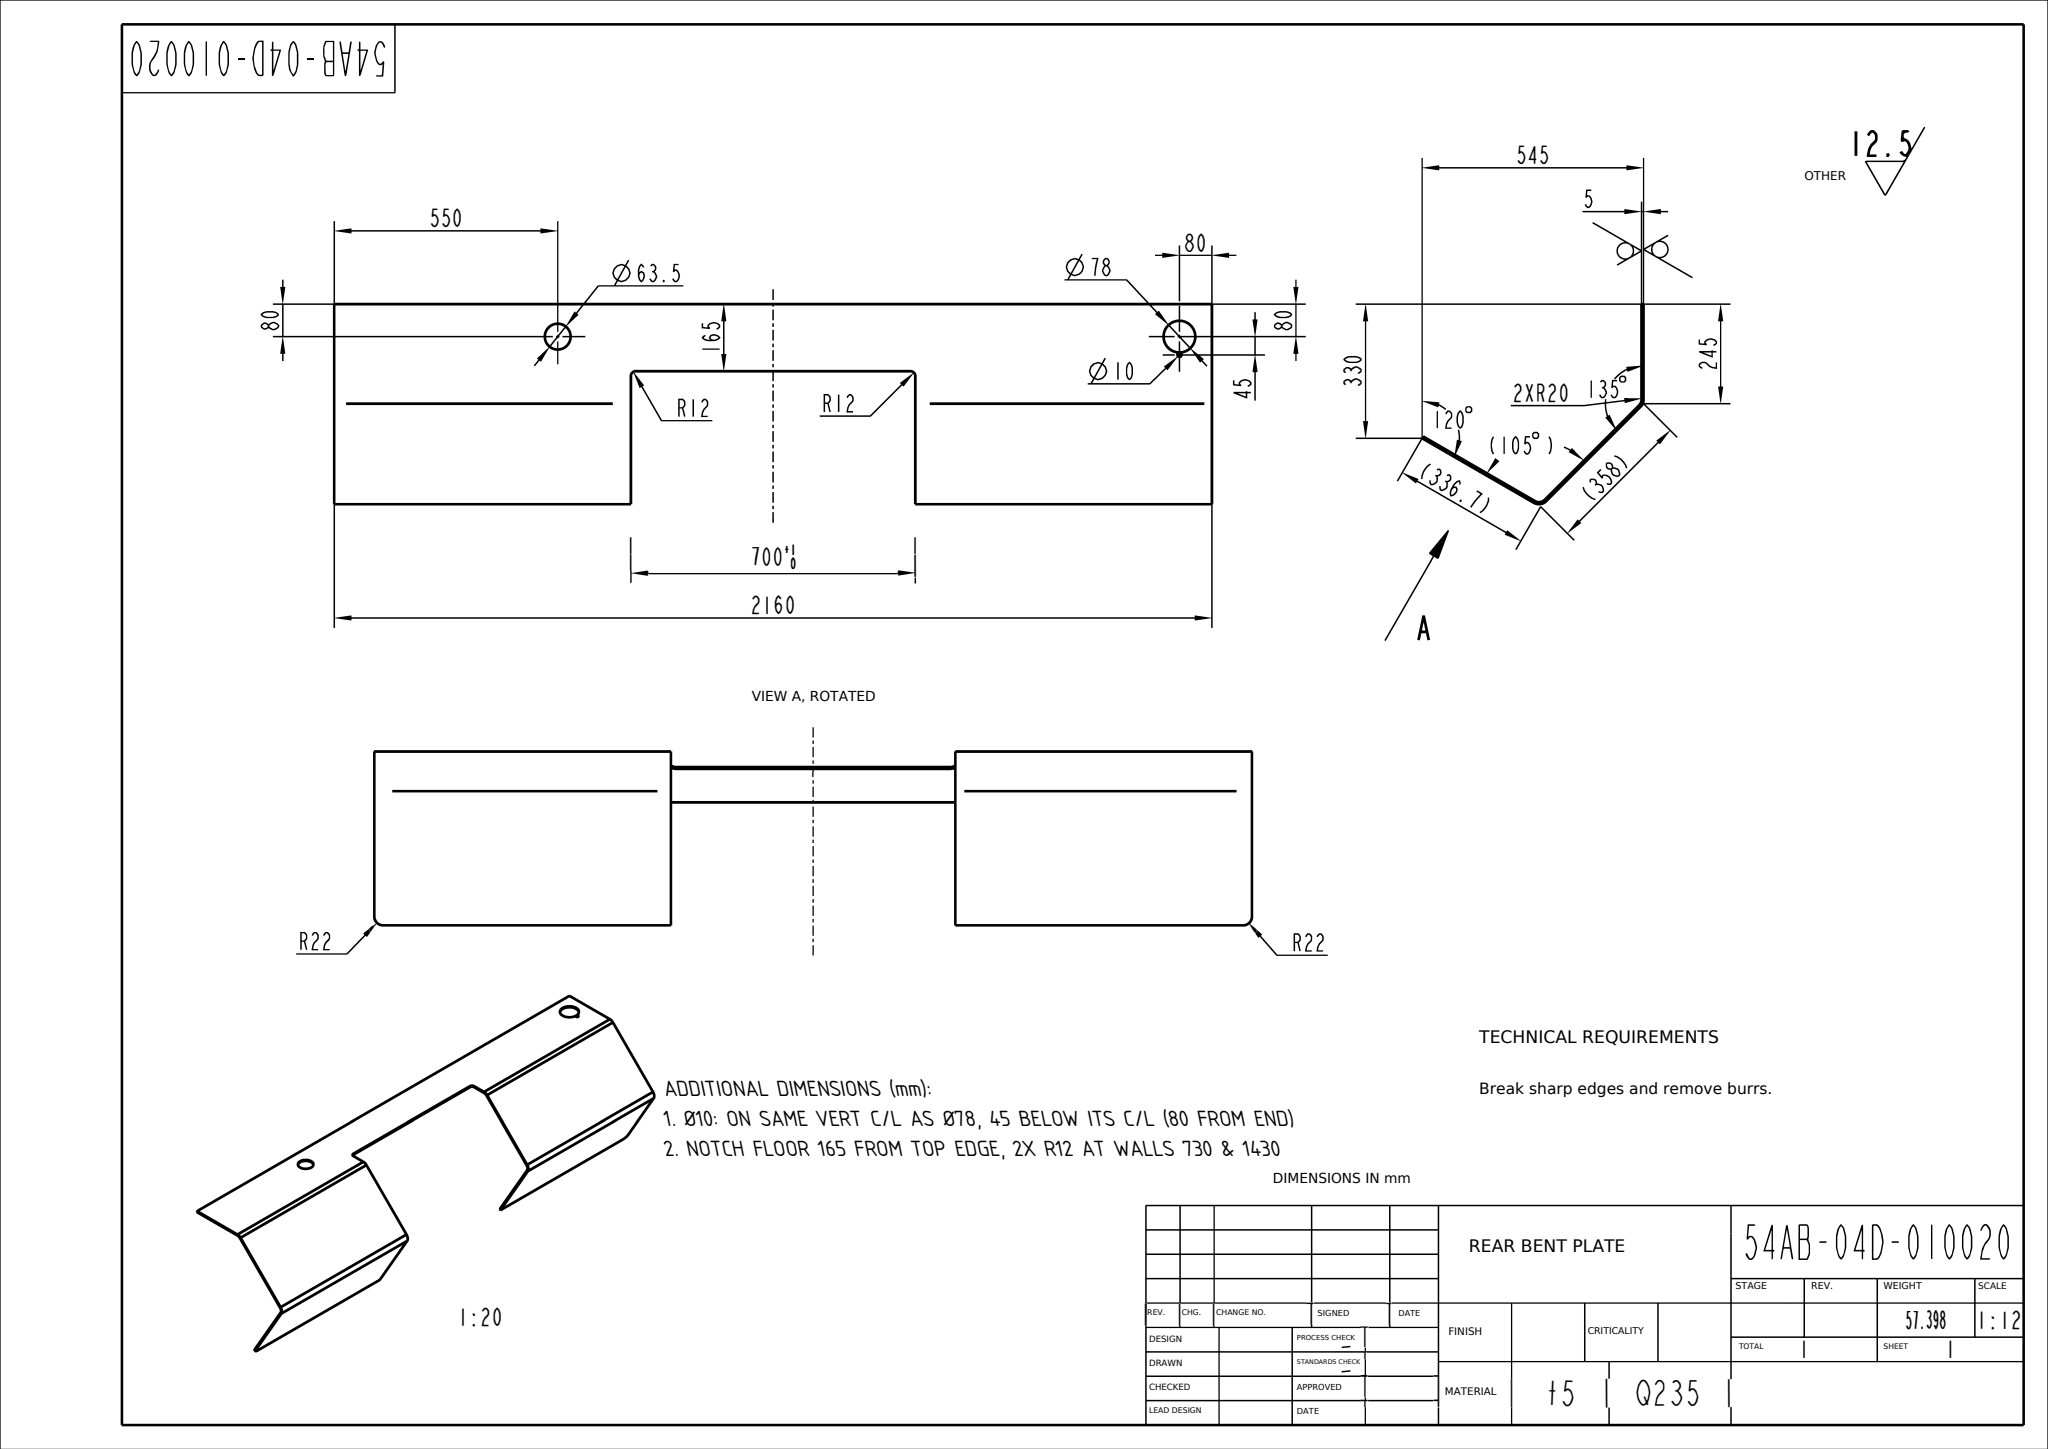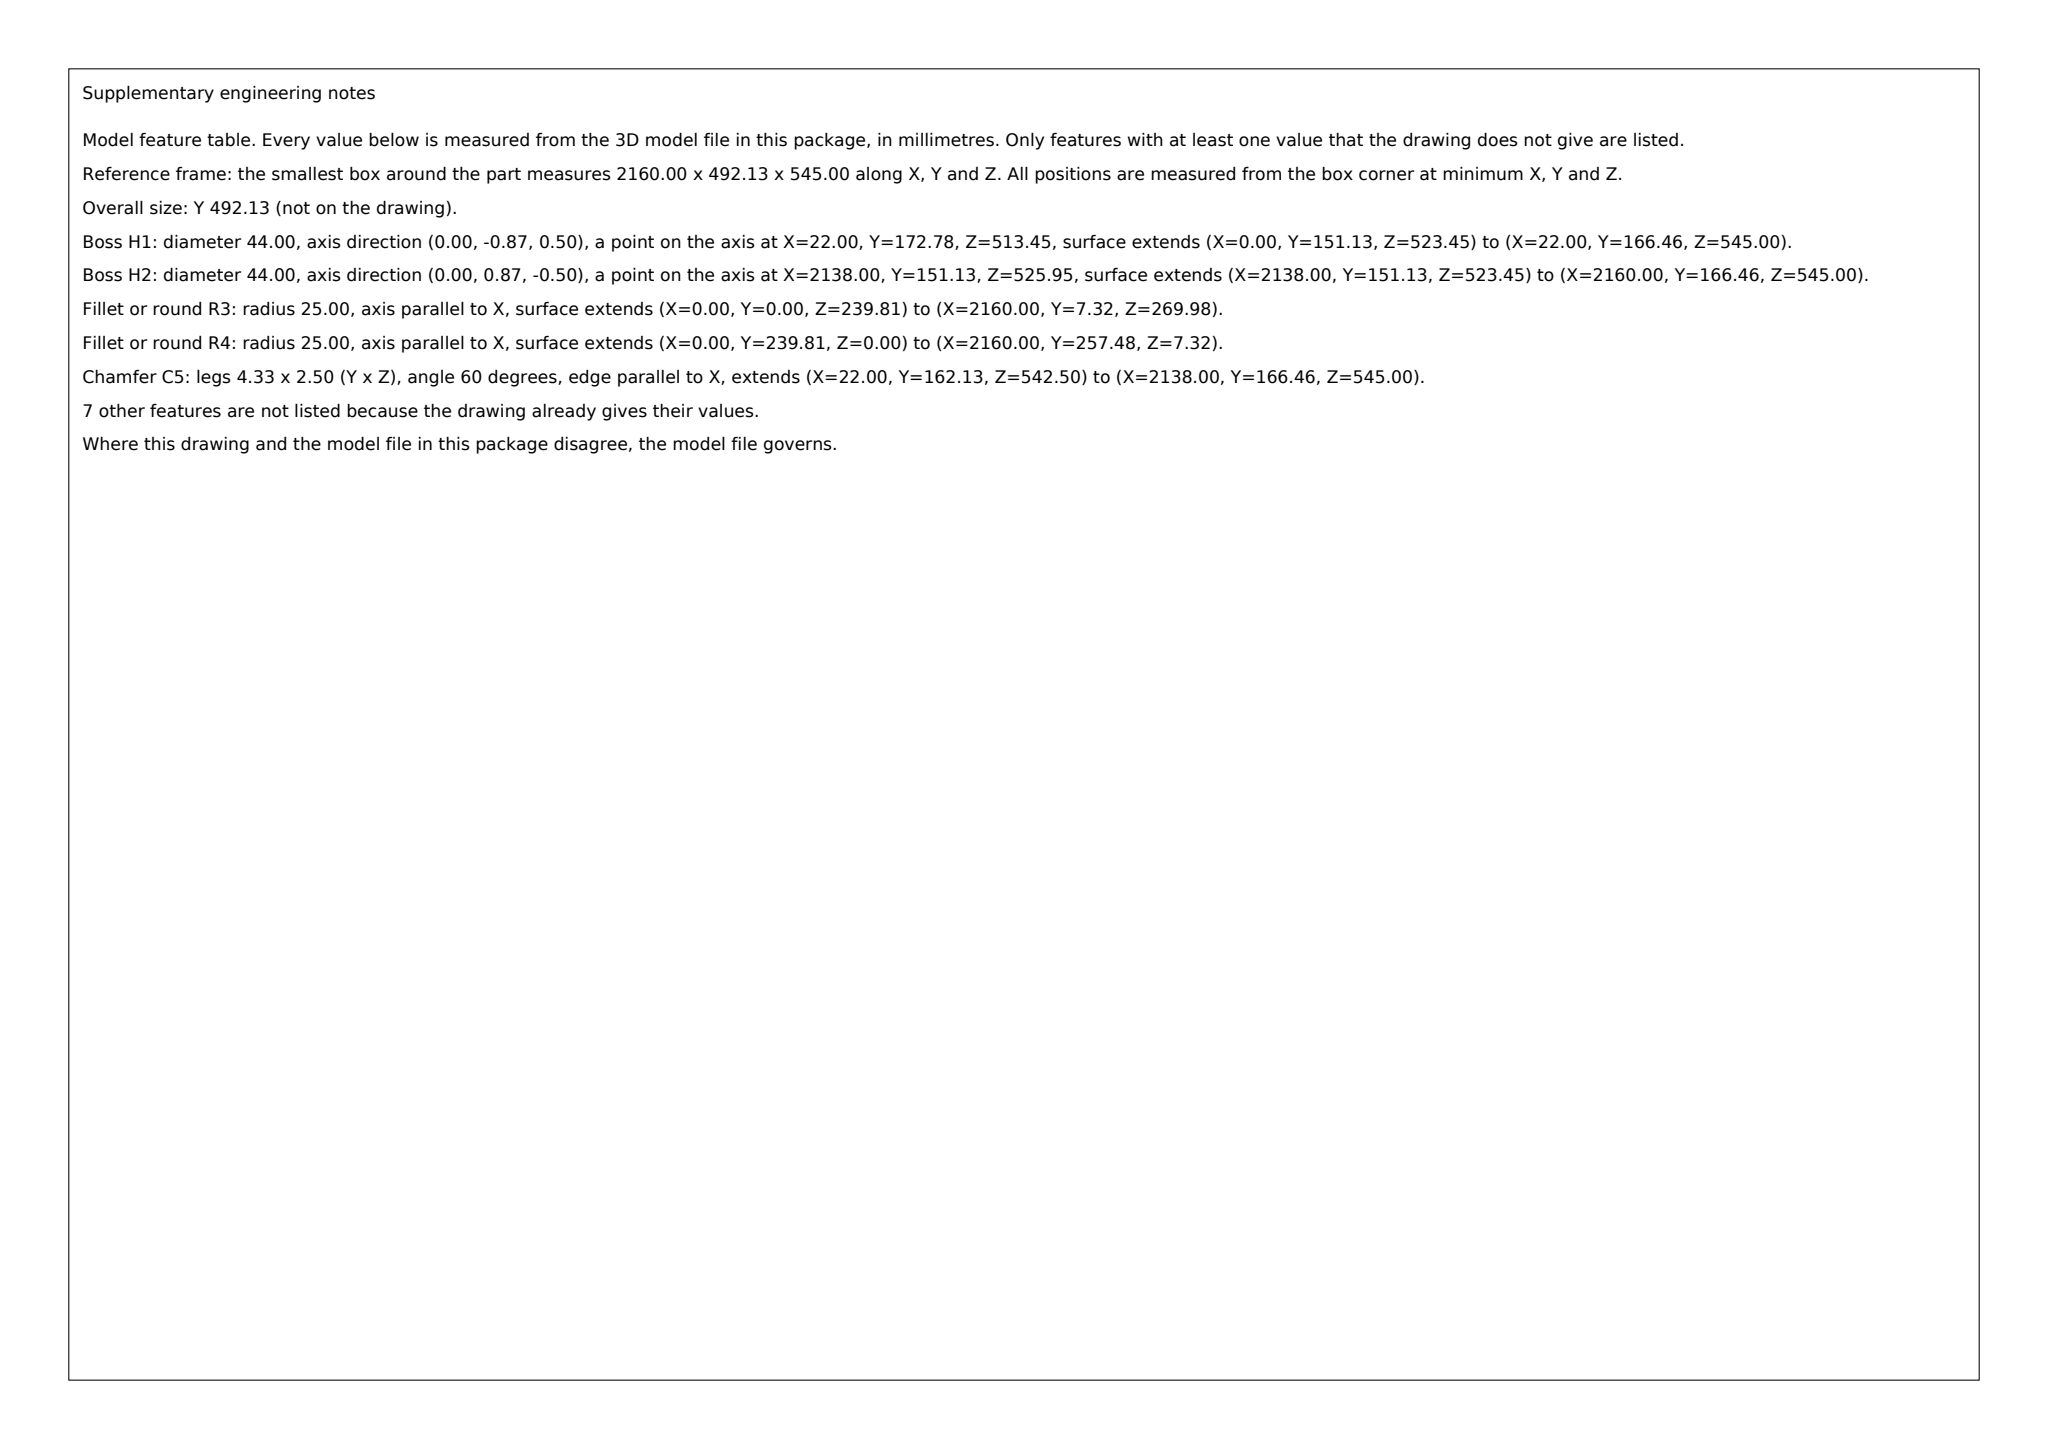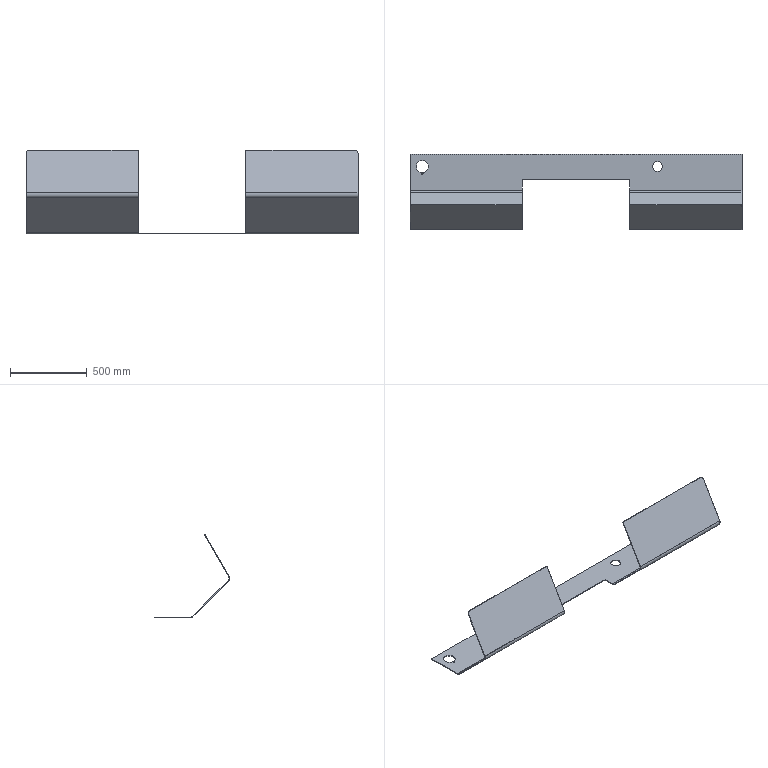Part | SolidWorks | mm | 1 solid | 52 faces | box 2160 x 492.13 x 545 mm | volume 7311868 mm3 | plane 34 | cylinder 18 | commonest cylinder face diameters 50 x4 40 x4 63.5 x2 10 x2 78 x2 24 x2 44 x2